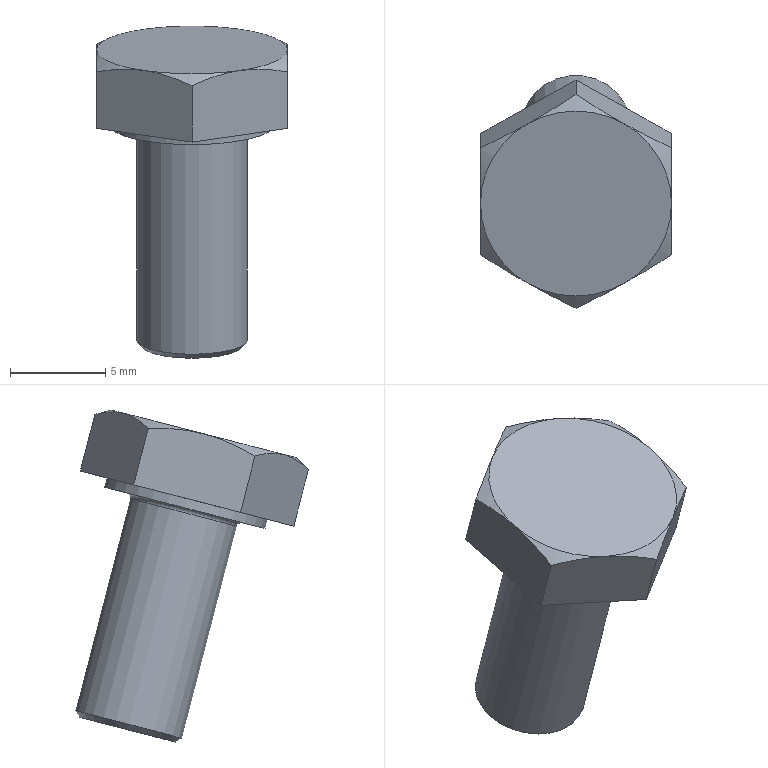Component | NX | GB-T5782-2000_M6X12 | 1 solid | 20 faces | volume 648 mm3 | plane 10 | cone 7 | cylinder 2 | torus 1 | commonest cylinder face diameters 8.74 x1 5.795 x1